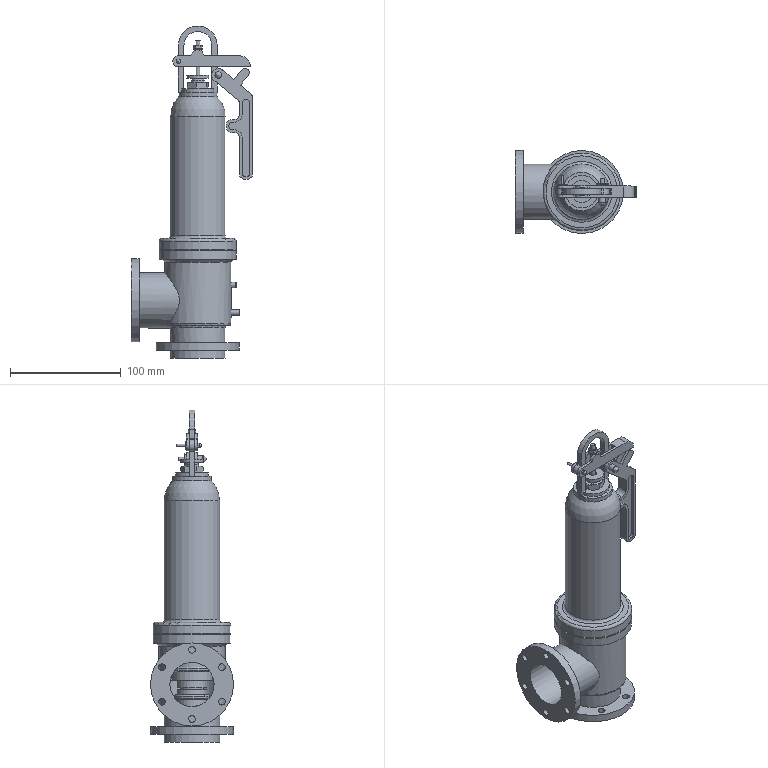Assembly | NX | mm | 25 component files | 25 solids | 406 faces | box 109.5 x 75 x 300 mm | volume 391352 mm3 | plane 179 | cylinder 134 | cone 66 | torus 21 | sphere 3 | spline 3 | commonest cylinder face diameters 6 x20 4 x19 12 x9 10 x8 5 x8 27 x7 20 x5 50 x5
Bill of materials:
unnamed part 1 | 1 |  | Hollow tee-shaped body. A large vertical cylindrical run has a side branch that ends in a flange, a bottom flange on a narrower neck, and a wider top rim with a stepped internal recess.
unnamed part 2 | 1 |  | Flat, uniformly thick plate bent into a U (hairpin) outline. Each leg has a round eyelet lug with a hole, and the two lugs sit at different heights.
unnamed part 3 | 1 |  | Flanged cylindrical bushing: a thin circular flange on top of a plain cylindrical shank, with a small central axial hole.
GB923_A-88,M4 | 1 |  | Hexagonal prism body with chamfered corner edges, joined to a closed domed (roughly hemispherical) end on one side; the opposite flat face has a central blind circular bore with a small chamfer or counterbore at its entry and a conical bottom. The shape matches an acorn/cap-nut style form.
unnamed part 4 | 2 |  | Half (D-section) of a stepped solid of revolution: a smaller upper cylinder, a larger cylindrical band, and a conical point at the bottom. The flat face has a semicircular notch on the axis.
GB-T848-2002,M4 | 1 |  | Thin flat annular disc (ring) with a concentric circular through-hole, uniform thickness and plain square edges. The shape matches a plain flat washer.
unnamed part 5 | 1 |  | Three-step cylindrical bushing: a thin wide base flange, a mid-diameter section, and a narrow top tube, with a central through bore chamfered at the top.
unnamed part 6 | 2 |  | Round disc with chamfered top and bottom outer edges, a shallow annular groove on one face, and a small central through hole.
unnamed part 7 | 1 |  | Open-wound cylindrical helical coil of round wire with many turns at roughly uniform pitch.
unnamed part 8 | 1 |  | Headed pin assembly shape: a cylindrical body with a domed end, a countersunk (conical) head at the other end, and a thinner rod projecting from the head side.
unnamed part 9 | 1 |  | Split circular band ring with rectangular overlapping/offset tabs at the gap.
unnamed part 10 | 1 |  | Solid cylindrical pin with chamfered ends; one end face shows a small polygonal recess.
unnamed part 11 | 1 |  | Flat lever-like bracket made of two parallel plates (clevis-style) joined by a block. It has an elongated rounded body, a side lobe midway, and a forked/branched upper end with a hole.
unnamed part 12 | 1 |  | Headed pin with a flat round head, a small undercut groove under the head, a cylindrical shank, and a conical pointed tip. A central hole with a chamfered entry is in the head.
unnamed part 13 | 1 |  | Long, slender cylindrical rod with a short, larger-diameter cylindrical collar near one end; a short small-diameter stub extends beyond the collar.
unnamed part 14 | 1 |  | Thin, flat split ring with a rectangular cross-section and rounded edges; the two ends overlap in a stepped, interlocking joint that sticks out slightly beyond the ring's outer diameter.
unnamed part 15 | 1 |  | Solid cylindrical pin with chamfered ends; one end face has a polygonal drive-socket recess and the other end face is plain and flat.
unnamed part 16 | 1 |  | Hollow cylindrical body with a flat flange at the base and a rounded shoulder at the top, which steps down to a small stepped boss with a central hole.
unnamed part 17 | 1 |  | Flat, elongated lever or link plate. One end is forked into a clevis by a slot through the thickness and has a cross hole. A rounded lobe rises from the top edge, and the opposite end is a large curved profile.
GB-T6170_F-2000,M4x0.7 | 1 |  | Hexagonal nut-shaped body with a central circular through-bore; both faces are chamfered and the bore entrance is chamfered or countersunk.
unnamed part 18 | 1 |  | Pin-like body with a cylindrical shank ending in a domed end, a conical countersunk-style head at the other end, and a smaller-diameter coaxial pin sticking out from the head.
unnamed part 19 | 1 |  | Tubular cylindrical sleeve with a central through-bore and three rectangular circumferential grooves along one end region; the remaining length is plain.
GB-T6172_1-2000,M12x1.75 | 1 |  | Hexagon Thin Nut, Chamfered, GB-T 6172.1-2000,M12x1.75
Mates:
1. touch align | Valve_Bonnet 1 face | Valve_Body 1 face
2. touch align | Lock_Pin 1 face | Valve_Body 1 face
3. touch align | Ejector_Pin 1 face | Valve_Body 1 face
4. touch align | Retaining_Ring 1 face | Valve_Bonnet 1 face
5. touch align | Mandrel 1 face | Valve_Bonnet 1 face
6. touch align | Retainer_Plate 1 face | Retaining_Ring 1 face
7. touch align | Retainer_Plate 1 face | Retaining_Ring 1 face
8. touch align | Handle 1 face | Retaining_Ring 1 face
9. touch align | Handle 1 face | Retaining_Ring 1 face
10. touch align | Collar 1 face | Mandrel 1 face
11. touch align | Base 1 face | Valve_Body 1 face
12. touch align | Base 1 face | Valve_Body 1 face
13. touch align | Clamp_2 1 face | Base 1 face
14. touch align | Shaft_Sleeve 1 face | Base 1 face
15. touch align | Shaft_Sleeve 1 face | Valve_Bonnet 1 face
16. touch align | Sleeve 1 face | Shaft_Sleeve 1 face
17. touch align | Valve_Disc 2 face | Sleeve 1 face
18. touch align | Spring_Seat 2 face | Collar 1 face
19. touch align | Pivot_Pin 1 face | Retaining_Ring 1 face
20. touch align | Dowel_Pin 1 face | Retainer_Plate 1 face
21. touch align | Nut_M4 1 face | Mandrel 1 face
22. touch align | Washer_M4 1 face | Mandrel 1 face
23. touch align | Nut_M12 1 face | Collar 1 face
24. touch align | Flange_Nut_M4 1 face | Mandrel 1 face